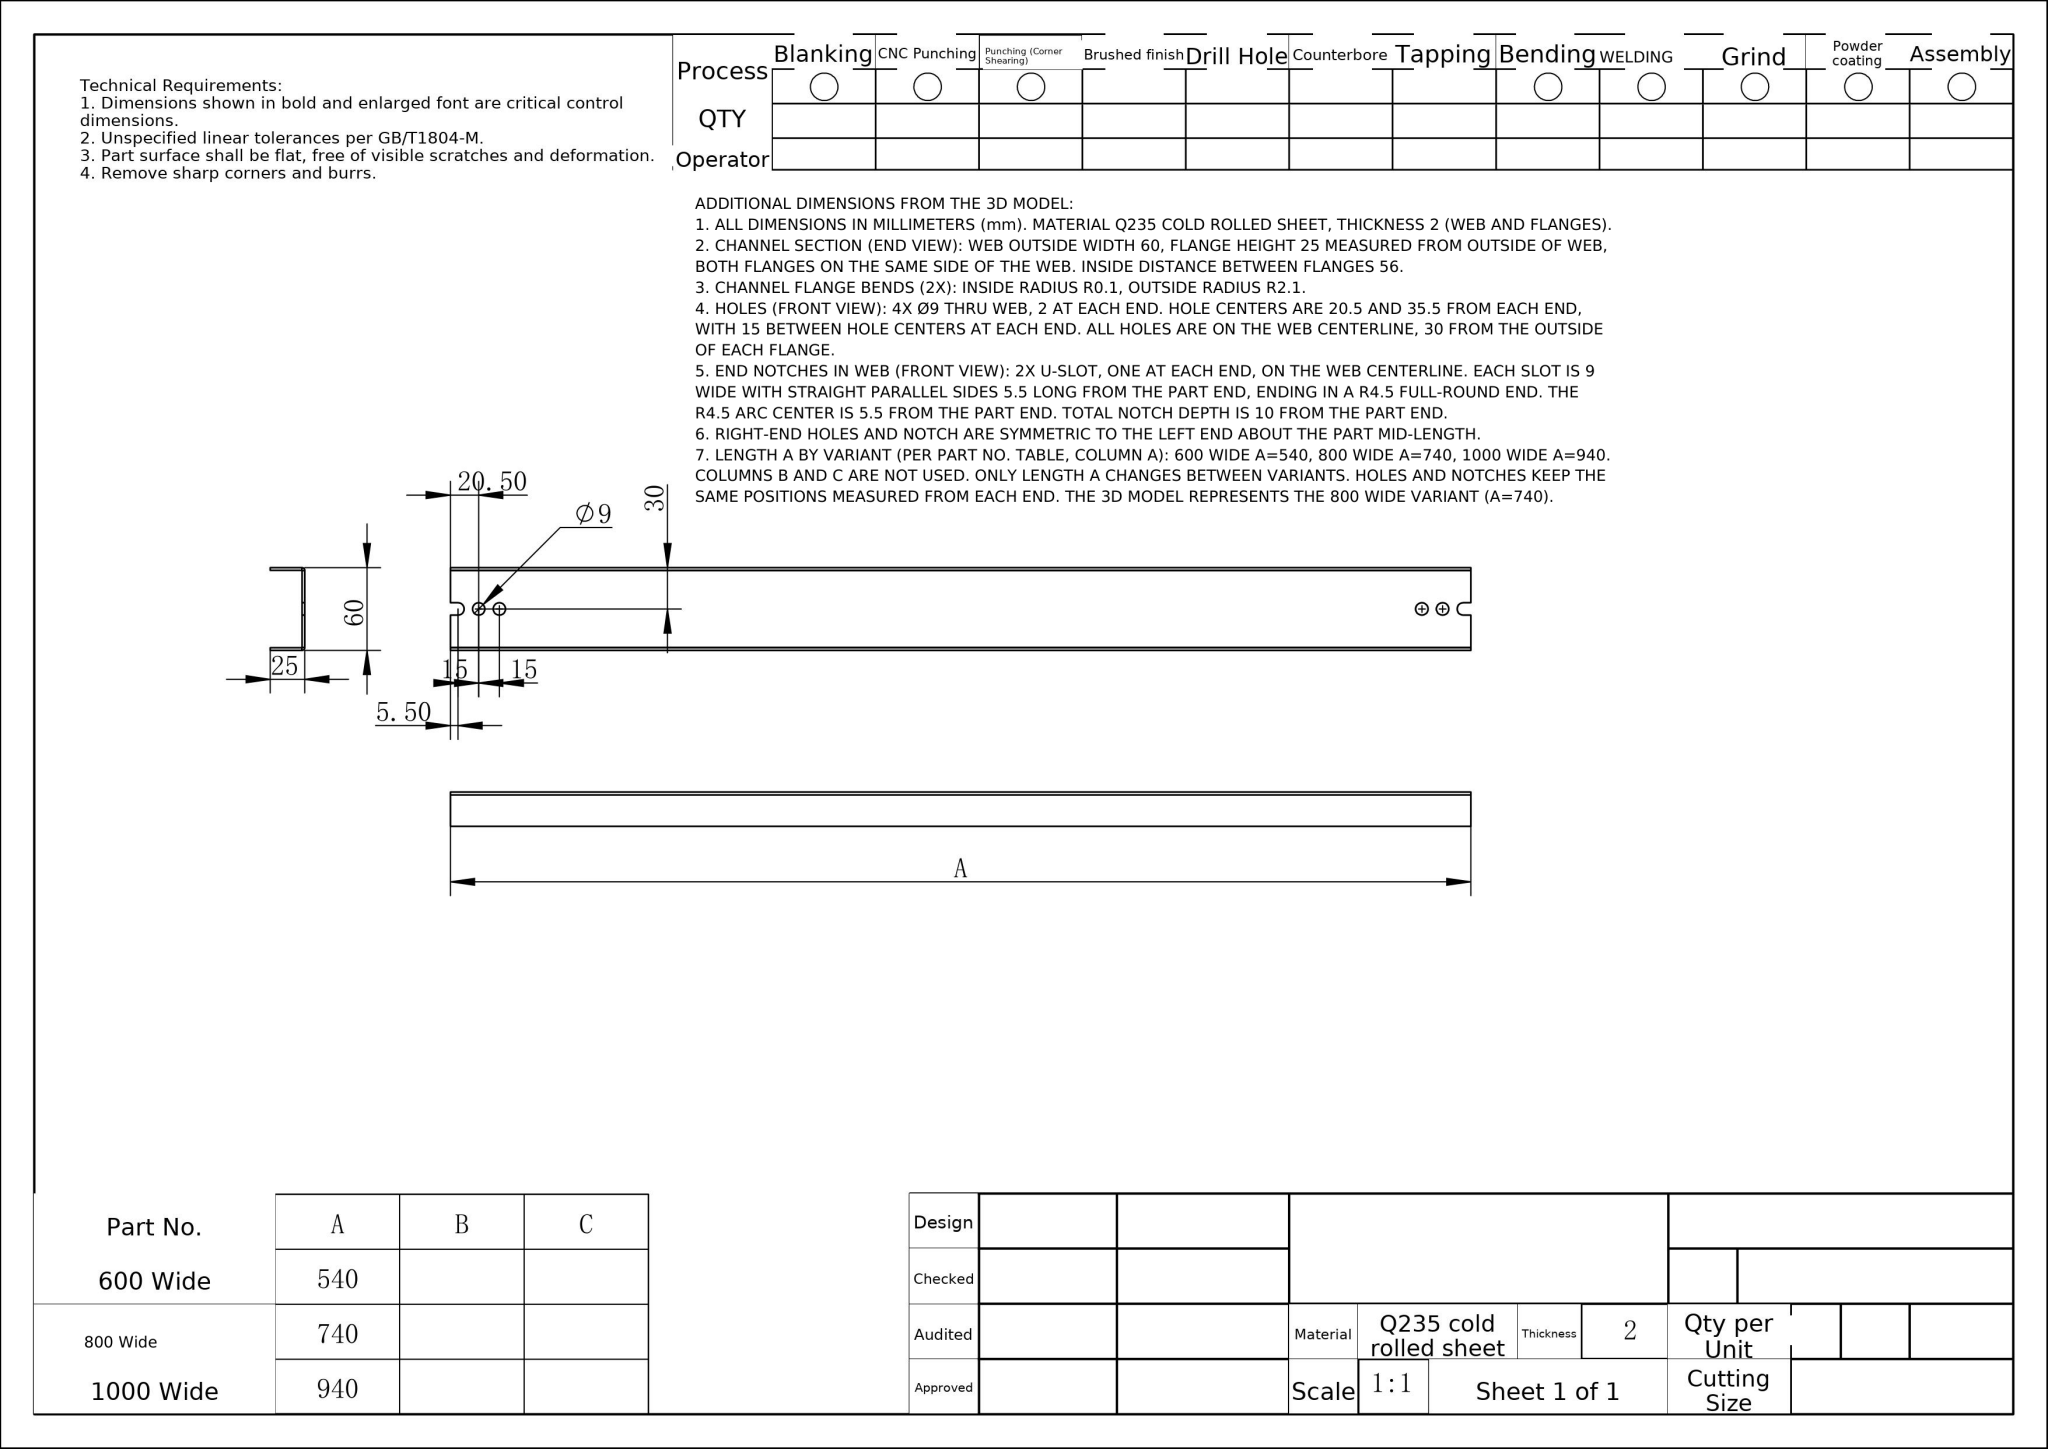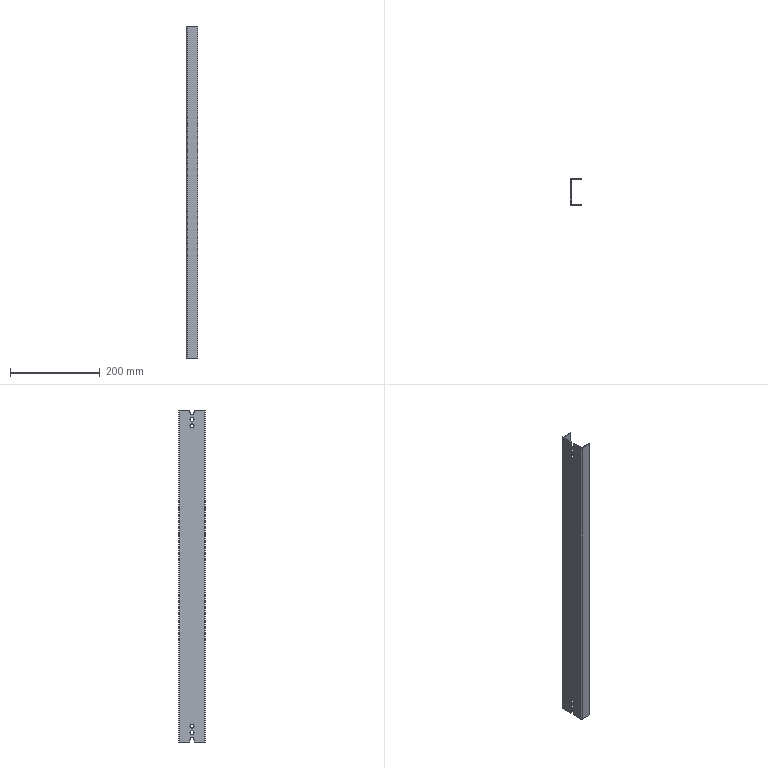Part | NX | mm | 1 solid | 38 faces | box 25 x 60 x 740 mm | volume 154648 mm3 | plane 24 | cylinder 14 | commonest cylinder face diameters 9 x10 4.2 x2 0.2 x2